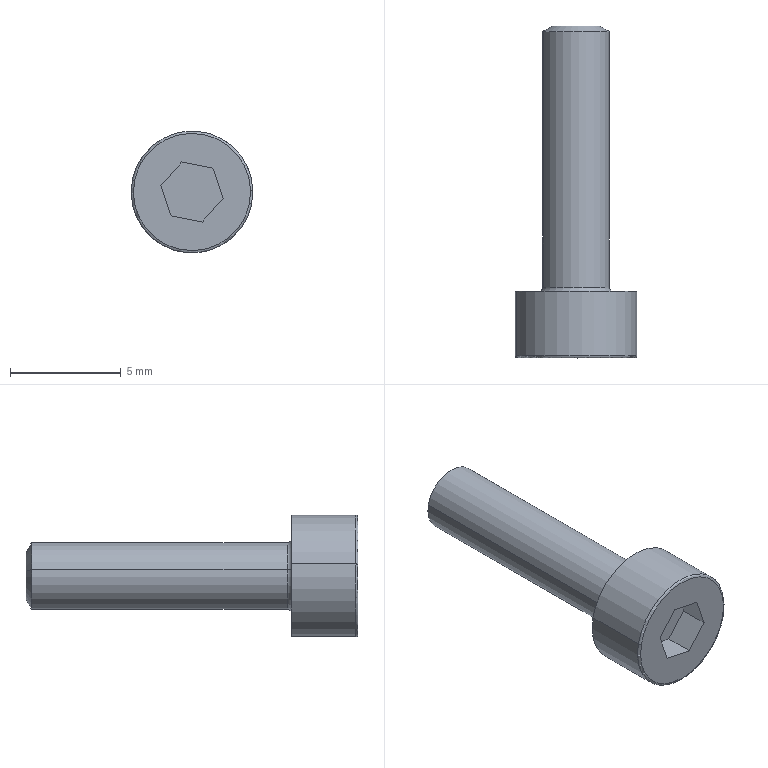Component | SolidWorks | MGL-PACK-01-00WeldedPlate1Assembly-1_SocketHeadCapScrew_M3_12[GB_T70.1-2000]-1 | 1 solid | 20 faces | box 5.5 x 15 x 5.5 mm | volume 149 mm3 | plane 10 | torus 4 | cylinder 4 | cone 2 | commonest cylinder face diameters 5.5 x2 3 x2
STEP:
#1=COLOUR_RGB('',0.7922,0.8196,0.9333);
#2=FILL_AREA_STYLE_COLOUR('',#1);
#3=FILL_AREA_STYLE('',(#2));
#4=SURFACE_STYLE_FILL_AREA(#3);
#5=SURFACE_SIDE_STYLE('',(#4));
#6=SURFACE_STYLE_USAGE(.BOTH.,#5);
#7=PRESENTATION_STYLE_ASSIGNMENT((#6));
#8=CARTESIAN_POINT('',(6.195,-2.224,0.3552));
#9=VERTEX_POINT('',#8);
#10=CARTESIAN_POINT('',(6.4,-2.224,0.314));
#11=VERTEX_POINT('',#10);
#12=CARTESIAN_POINT('',(6.297,-2.224,0.3346));
#13=DIRECTION('',(0.,-1.,-0.));
#14=DIRECTION('',(0.9803,0.,-0.1975));
#15=AXIS2_PLACEMENT_3D('',#12,#13,#14);
#16=CIRCLE('',#15,0.1043);
#17=EDGE_CURVE('',#9,#11,#16,.T.);
#18=ORIENTED_EDGE('',*,*,#17,.F.);
#19=CARTESIAN_POINT('',(6.191,-2.22,0.356));
#20=VERTEX_POINT('',#19);
#21=CARTESIAN_POINT('',(6.195,-2.22,0.3552));
#22=DIRECTION('',(-0.1975,0.,-0.9803));
#23=DIRECTION('',(-0.9803,0.,0.1975));
#24=AXIS2_PLACEMENT_3D('',#21,#22,#23);
#25=CIRCLE('',#24,0.003937);
#26=EDGE_CURVE('',#9,#20,#25,.T.);
#27=ORIENTED_EDGE('',*,*,#26,.T.);
#28=CARTESIAN_POINT('',(6.403,-2.22,0.3133));
#29=VERTEX_POINT('',#28);
#30=CARTESIAN_POINT('',(6.297,-2.22,0.3346));
#31=DIRECTION('',(-0.,1.,0.));
#32=DIRECTION('',(0.9803,0.,-0.1975));
#33=AXIS2_PLACEMENT_3D('',#30,#31,#32);
#34=CIRCLE('',#33,0.1083);
#35=EDGE_CURVE('',#29,#20,#34,.T.);
#36=ORIENTED_EDGE('',*,*,#35,.F.);
#37=CARTESIAN_POINT('',(6.4,-2.22,0.314));
#38=DIRECTION('',(0.1975,-0.,0.9803));
#39=DIRECTION('',(0.9803,0.,-0.1975));
#40=AXIS2_PLACEMENT_3D('',#37,#38,#39);
#41=CIRCLE('',#40,0.003937);
#42=EDGE_CURVE('',#11,#29,#41,.T.);
#43=ORIENTED_EDGE('',*,*,#42,.F.);
#44=EDGE_LOOP('',(#18,#27,#36,#43));
#45=FACE_OUTER_BOUND('',#44,.T.);
#46=CARTESIAN_POINT('',(6.297,-2.22,0.3346));
#47=DIRECTION('',(-0.,1.,0.));
#48=DIRECTION('',(0.9803,0.,-0.1975));
#49=AXIS2_PLACEMENT_3D('',#46,#47,#48);
#50=TOROIDAL_SURFACE('',#49,0.1043,0.003937);
#51=ADVANCED_FACE('',(#45),#50,.T.);
#52=CARTESIAN_POINT('',(6.256,-1.634,0.3429));
#53=VERTEX_POINT('',#52);
#54=CARTESIAN_POINT('',(6.338,-1.634,0.3264));
#55=VERTEX_POINT('',#54);
#56=CARTESIAN_POINT('',(6.297,-1.634,0.3346));
#57=DIRECTION('',(0.,-1.,-0.));
#58=DIRECTION('',(-0.9803,0.,0.1975));
#59=AXIS2_PLACEMENT_3D('',#56,#57,#58);
#60=CIRCLE('',#59,0.04201);
#61=EDGE_CURVE('',#53,#55,#60,.T.);
#62=ORIENTED_EDGE('',*,*,#61,.T.);
#63=CARTESIAN_POINT('',(6.355,-1.644,0.323));
#64=VERTEX_POINT('',#63);
#65=CARTESIAN_POINT('',(6.355,-1.644,0.323));
#66=DIRECTION('',(0.849,-0.5,-0.171));
#67=VECTOR('',#66,39.37);
#68=LINE('',#65,#67);
#69=EDGE_CURVE('',#55,#64,#68,.T.);
#70=ORIENTED_EDGE('',*,*,#69,.T.);
#71=CARTESIAN_POINT('',(6.239,-1.644,0.3463));
#72=VERTEX_POINT('',#71);
#73=CARTESIAN_POINT('',(6.297,-1.644,0.3346));
#74=DIRECTION('',(0.,-1.,-0.));
#75=DIRECTION('',(-0.9803,0.,0.1975));
#76=AXIS2_PLACEMENT_3D('',#73,#74,#75);
#77=CIRCLE('',#76,0.05906);
#78=EDGE_CURVE('',#72,#64,#77,.T.);
#79=ORIENTED_EDGE('',*,*,#78,.F.);
#80=CARTESIAN_POINT('',(6.239,-1.644,0.3463));
#81=DIRECTION('',(-0.849,-0.5,0.171));
#82=VECTOR('',#81,39.37);
#83=LINE('',#80,#82);
#84=EDGE_CURVE('',#53,#72,#83,.T.);
#85=ORIENTED_EDGE('',*,*,#84,.F.);
#86=EDGE_LOOP('',(#62,#70,#79,#85));
#87=FACE_OUTER_BOUND('',#86,.T.);
#88=CARTESIAN_POINT('',(6.297,-1.644,0.3346));
#89=DIRECTION('',(0.,-1.,-0.));
#90=DIRECTION('',(-0.9803,0.,0.1975));
#91=AXIS2_PLACEMENT_3D('',#88,#89,#90);
#92=CONICAL_SURFACE('',#91,0.05906,1.047);
#93=ADVANCED_FACE('',(#87),#92,.T.);
#94=CARTESIAN_POINT('',(6.363,-2.106,0.3214));
#95=VERTEX_POINT('',#94);
#96=CARTESIAN_POINT('',(6.232,-2.106,0.3479));
#97=VERTEX_POINT('',#96);
#98=CARTESIAN_POINT('',(6.297,-2.106,0.3346));
#99=DIRECTION('',(0.,-1.,-0.));
#100=DIRECTION('',(-0.9803,0.,0.1975));
#101=AXIS2_PLACEMENT_3D('',#98,#99,#100);
#102=CIRCLE('',#101,0.06693);
#103=EDGE_CURVE('',#95,#97,#102,.T.);
#104=ORIENTED_EDGE('',*,*,#103,.F.);
#105=CARTESIAN_POINT('',(6.355,-2.098,0.323));
#106=VERTEX_POINT('',#105);
#107=CARTESIAN_POINT('',(6.363,-2.098,0.3214));
#108=DIRECTION('',(-0.1975,0.,-0.9803));
#109=DIRECTION('',(-0.9803,0.,0.1975));
#110=AXIS2_PLACEMENT_3D('',#107,#108,#109);
#111=CIRCLE('',#110,0.007874);
#112=EDGE_CURVE('',#95,#106,#111,.T.);
#113=ORIENTED_EDGE('',*,*,#112,.T.);
#114=CARTESIAN_POINT('',(6.239,-2.098,0.3463));
#115=VERTEX_POINT('',#114);
#116=CARTESIAN_POINT('',(6.297,-2.098,0.3346));
#117=DIRECTION('',(0.,-1.,-0.));
#118=DIRECTION('',(-0.9803,0.,0.1975));
#119=AXIS2_PLACEMENT_3D('',#116,#117,#118);
#120=CIRCLE('',#119,0.05906);
#121=EDGE_CURVE('',#106,#115,#120,.T.);
#122=ORIENTED_EDGE('',*,*,#121,.T.);
#123=CARTESIAN_POINT('',(6.232,-2.098,0.3479));
#124=DIRECTION('',(0.1975,-0.,0.9803));
#125=DIRECTION('',(0.9803,0.,-0.1975));
#126=AXIS2_PLACEMENT_3D('',#123,#124,#125);
#127=CIRCLE('',#126,0.007874);
#128=EDGE_CURVE('',#97,#115,#127,.T.);
#129=ORIENTED_EDGE('',*,*,#128,.F.);
#130=EDGE_LOOP('',(#104,#113,#122,#129));
#131=FACE_OUTER_BOUND('',#130,.T.);
#132=CARTESIAN_POINT('',(6.297,-2.098,0.3346));
#133=DIRECTION('',(0.,-1.,-0.));
#134=DIRECTION('',(-0.9803,-0.,0.1975));
#135=AXIS2_PLACEMENT_3D('',#132,#133,#134);
#136=TOROIDAL_SURFACE('',#135,0.06693,0.007874);
#137=ADVANCED_FACE('',(#131),#136,.F.);
#138=CARTESIAN_POINT('',(6.191,-2.106,0.356));
#139=VERTEX_POINT('',#138);
#140=CARTESIAN_POINT('',(6.403,-2.106,0.3133));
#141=VERTEX_POINT('',#140);
#142=CARTESIAN_POINT('',(6.297,-2.106,0.3346));
#143=DIRECTION('',(0.,-1.,-0.));
#144=DIRECTION('',(-0.9803,0.,0.1975));
#145=AXIS2_PLACEMENT_3D('',#142,#143,#144);
#146=CIRCLE('',#145,0.1083);
#147=EDGE_CURVE('',#139,#141,#146,.T.);
#148=ORIENTED_EDGE('',*,*,#147,.T.);
#149=CARTESIAN_POINT('',(6.403,-2.224,0.3133));
#150=DIRECTION('',(0.,-1.,-0.));
#151=VECTOR('',#150,39.37);
#152=LINE('',#149,#151);
#153=EDGE_CURVE('',#141,#29,#152,.T.);
#154=ORIENTED_EDGE('',*,*,#153,.T.);
#155=ORIENTED_EDGE('',*,*,#35,.T.);
#156=CARTESIAN_POINT('',(6.191,-2.224,0.356));
#157=DIRECTION('',(0.,-1.,-0.));
#158=VECTOR('',#157,39.37);
#159=LINE('',#156,#158);
#160=EDGE_CURVE('',#139,#20,#159,.T.);
#161=ORIENTED_EDGE('',*,*,#160,.F.);
#162=EDGE_LOOP('',(#148,#154,#155,#161));
#163=FACE_OUTER_BOUND('',#162,.T.);
#164=CARTESIAN_POINT('',(6.297,-2.224,0.3346));
#165=DIRECTION('',(0.,-1.,-0.));
#166=DIRECTION('',(-0.9803,0.,0.1975));
#167=AXIS2_PLACEMENT_3D('',#164,#165,#166);
#168=CYLINDRICAL_SURFACE('',#167,0.1083);
#169=ADVANCED_FACE('',(#163),#168,.T.);
#170=ORIENTED_EDGE('',*,*,#78,.T.);
#171=CARTESIAN_POINT('',(6.355,-2.224,0.323));
#172=DIRECTION('',(0.,-1.,-0.));
#173=VECTOR('',#172,39.37);
#174=LINE('',#171,#173);
#175=EDGE_CURVE('',#64,#106,#174,.T.);
#176=ORIENTED_EDGE('',*,*,#175,.T.);
#177=CARTESIAN_POINT('',(6.297,-2.098,0.3346));
#178=DIRECTION('',(0.,-1.,-0.));
#179=DIRECTION('',(-0.9803,0.,0.1975));
#180=AXIS2_PLACEMENT_3D('',#177,#178,#179);
#181=CIRCLE('',#180,0.05906);
#182=EDGE_CURVE('',#115,#106,#181,.T.);
#183=ORIENTED_EDGE('',*,*,#182,.F.);
#184=CARTESIAN_POINT('',(6.239,-2.224,0.3463));
#185=DIRECTION('',(0.,-1.,-0.));
#186=VECTOR('',#185,39.37);
#187=LINE('',#184,#186);
#188=EDGE_CURVE('',#72,#115,#187,.T.);
#189=ORIENTED_EDGE('',*,*,#188,.F.);
#190=EDGE_LOOP('',(#170,#176,#183,#189));
#191=FACE_OUTER_BOUND('',#190,.T.);
#192=CARTESIAN_POINT('',(6.297,-2.224,0.3346));
#193=DIRECTION('',(0.,-1.,-0.));
#194=DIRECTION('',(-0.9803,0.,0.1975));
#195=AXIS2_PLACEMENT_3D('',#192,#193,#194);
#196=CYLINDRICAL_SURFACE('',#195,0.05906);
#197=ADVANCED_FACE('',(#191),#196,.T.);
#198=ORIENTED_EDGE('',*,*,#175,.F.);
#199=CARTESIAN_POINT('',(6.297,-1.644,0.3346));
#200=DIRECTION('',(0.,-1.,-0.));
#201=DIRECTION('',(-0.9803,0.,0.1975));
#202=AXIS2_PLACEMENT_3D('',#199,#200,#201);
#203=CIRCLE('',#202,0.05906);
#204=EDGE_CURVE('',#64,#72,#203,.T.);
#205=ORIENTED_EDGE('',*,*,#204,.T.);
#206=ORIENTED_EDGE('',*,*,#188,.T.);
#207=ORIENTED_EDGE('',*,*,#121,.F.);
#208=EDGE_LOOP('',(#198,#205,#206,#207));
#209=FACE_OUTER_BOUND('',#208,.T.);
#210=CARTESIAN_POINT('',(6.297,-2.224,0.3346));
#211=DIRECTION('',(0.,-1.,-0.));
#212=DIRECTION('',(-0.9803,0.,0.1975));
#213=AXIS2_PLACEMENT_3D('',#210,#211,#212);
#214=CYLINDRICAL_SURFACE('',#213,0.05906);
#215=ADVANCED_FACE('',(#209),#214,.T.);
#216=CARTESIAN_POINT('',(6.297,-2.224,0.3346));
#217=DIRECTION('',(0.,-1.,-0.));
#218=DIRECTION('',(0.9803,0.,-0.1975));
#219=AXIS2_PLACEMENT_3D('',#216,#217,#218);
#220=CIRCLE('',#219,0.1043);
#221=EDGE_CURVE('',#11,#9,#220,.T.);
#222=ORIENTED_EDGE('',*,*,#221,.T.);
#223=ORIENTED_EDGE('',*,*,#17,.T.);
#224=EDGE_LOOP('',(#222,#223));
#225=FACE_OUTER_BOUND('',#224,.T.);
#226=CARTESIAN_POINT('',(6.242,-2.224,0.3458));
#227=VERTEX_POINT('',#226);
#228=CARTESIAN_POINT('',(6.26,-2.224,0.2923));
#229=VERTEX_POINT('',#228);
#230=CARTESIAN_POINT('',(6.242,-2.224,0.3458));
#231=DIRECTION('',(0.3192,0.,-0.9477));
#232=VECTOR('',#231,39.37);
#233=LINE('',#230,#232);
#234=EDGE_CURVE('',#227,#229,#233,.T.);
#235=ORIENTED_EDGE('',*,*,#234,.F.);
#236=CARTESIAN_POINT('',(6.279,-2.224,0.3882));
#237=VERTEX_POINT('',#236);
#238=CARTESIAN_POINT('',(6.279,-2.224,0.3882));
#239=DIRECTION('',(-0.6612,0.,-0.7502));
#240=VECTOR('',#239,39.37);
#241=LINE('',#238,#240);
#242=EDGE_CURVE('',#237,#227,#241,.T.);
#243=ORIENTED_EDGE('',*,*,#242,.F.);
#244=CARTESIAN_POINT('',(6.335,-2.224,0.377));
#245=VERTEX_POINT('',#244);
#246=CARTESIAN_POINT('',(6.335,-2.224,0.377));
#247=DIRECTION('',(-0.9803,-0.,0.1975));
#248=VECTOR('',#247,39.37);
#249=LINE('',#246,#248);
#250=EDGE_CURVE('',#245,#237,#249,.T.);
#251=ORIENTED_EDGE('',*,*,#250,.F.);
#252=CARTESIAN_POINT('',(6.353,-2.224,0.3235));
#253=VERTEX_POINT('',#252);
#254=CARTESIAN_POINT('',(6.353,-2.224,0.3235));
#255=DIRECTION('',(-0.3192,-0.,0.9477));
#256=VECTOR('',#255,39.37);
#257=LINE('',#254,#256);
#258=EDGE_CURVE('',#253,#245,#257,.T.);
#259=ORIENTED_EDGE('',*,*,#258,.F.);
#260=CARTESIAN_POINT('',(6.315,-2.224,0.2811));
#261=VERTEX_POINT('',#260);
#262=CARTESIAN_POINT('',(6.315,-2.224,0.2811));
#263=DIRECTION('',(0.6612,-0.,0.7502));
#264=VECTOR('',#263,39.37);
#265=LINE('',#262,#264);
#266=EDGE_CURVE('',#261,#253,#265,.T.);
#267=ORIENTED_EDGE('',*,*,#266,.F.);
#268=CARTESIAN_POINT('',(6.26,-2.224,0.2923));
#269=DIRECTION('',(0.9803,0.,-0.1975));
#270=VECTOR('',#269,39.37);
#271=LINE('',#268,#270);
#272=EDGE_CURVE('',#229,#261,#271,.T.);
#273=ORIENTED_EDGE('',*,*,#272,.F.);
#274=EDGE_LOOP('',(#235,#243,#251,#259,#267,#273));
#275=FACE_BOUND('',#274,.T.);
#276=CARTESIAN_POINT('',(6.297,-2.224,0.3346));
#277=DIRECTION('',(-0.,1.,0.));
#278=DIRECTION('',(0.9803,0.,-0.1975));
#279=AXIS2_PLACEMENT_3D('',#276,#277,#278);
#280=PLANE('',#279);
#281=ADVANCED_FACE('',(#225,#275),#280,.F.);
#282=ORIENTED_EDGE('',*,*,#153,.F.);
#283=CARTESIAN_POINT('',(6.297,-2.106,0.3346));
#284=DIRECTION('',(0.,-1.,-0.));
#285=DIRECTION('',(-0.9803,0.,0.1975));
#286=AXIS2_PLACEMENT_3D('',#283,#284,#285);
#287=CIRCLE('',#286,0.1083);
#288=EDGE_CURVE('',#141,#139,#287,.T.);
#289=ORIENTED_EDGE('',*,*,#288,.T.);
#290=ORIENTED_EDGE('',*,*,#160,.T.);
#291=CARTESIAN_POINT('',(6.297,-2.22,0.3346));
#292=DIRECTION('',(-0.,1.,0.));
#293=DIRECTION('',(0.9803,0.,-0.1975));
#294=AXIS2_PLACEMENT_3D('',#291,#292,#293);
#295=CIRCLE('',#294,0.1083);
#296=EDGE_CURVE('',#20,#29,#295,.T.);
#297=ORIENTED_EDGE('',*,*,#296,.T.);
#298=EDGE_LOOP('',(#282,#289,#290,#297));
#299=FACE_OUTER_BOUND('',#298,.T.);
#300=CARTESIAN_POINT('',(6.297,-2.224,0.3346));
#301=DIRECTION('',(0.,-1.,-0.));
#302=DIRECTION('',(-0.9803,0.,0.1975));
#303=AXIS2_PLACEMENT_3D('',#300,#301,#302);
#304=CYLINDRICAL_SURFACE('',#303,0.1083);
#305=ADVANCED_FACE('',(#299),#304,.T.);
#306=ORIENTED_EDGE('',*,*,#147,.F.);
#307=ORIENTED_EDGE('',*,*,#288,.F.);
#308=EDGE_LOOP('',(#306,#307));
#309=FACE_OUTER_BOUND('',#308,.T.);
#310=CARTESIAN_POINT('',(6.297,-2.106,0.3346));
#311=DIRECTION('',(0.,-1.,-0.));
#312=DIRECTION('',(-0.9803,0.,0.1975));
#313=AXIS2_PLACEMENT_3D('',#310,#311,#312);
#314=CIRCLE('',#313,0.06693);
#315=EDGE_CURVE('',#97,#95,#314,.T.);
#316=ORIENTED_EDGE('',*,*,#315,.T.);
#317=ORIENTED_EDGE('',*,*,#103,.T.);
#318=EDGE_LOOP('',(#316,#317));
#319=FACE_BOUND('',#318,.T.);
#320=CARTESIAN_POINT('',(6.276,-2.106,0.2285));
#321=DIRECTION('',(0.,-1.,-0.));
#322=DIRECTION('',(-0.9803,-0.,0.1975));
#323=AXIS2_PLACEMENT_3D('',#320,#321,#322);
#324=PLANE('',#323);
#325=ADVANCED_FACE('',(#309,#319),#324,.F.);
#326=ORIENTED_EDGE('',*,*,#112,.F.);
#327=ORIENTED_EDGE('',*,*,#315,.F.);
#328=ORIENTED_EDGE('',*,*,#128,.T.);
#329=ORIENTED_EDGE('',*,*,#182,.T.);
#330=EDGE_LOOP('',(#326,#327,#328,#329));
#331=FACE_OUTER_BOUND('',#330,.T.);
#332=CARTESIAN_POINT('',(6.297,-2.098,0.3346));
#333=DIRECTION('',(0.,-1.,-0.));
#334=DIRECTION('',(-0.9803,-0.,0.1975));
#335=AXIS2_PLACEMENT_3D('',#332,#333,#334);
#336=TOROIDAL_SURFACE('',#335,0.06693,0.007874);
#337=ADVANCED_FACE('',(#331),#336,.F.);
#338=ORIENTED_EDGE('',*,*,#242,.T.);
#339=CARTESIAN_POINT('',(6.242,-2.173,0.3458));
#340=VERTEX_POINT('',#339);
#341=CARTESIAN_POINT('',(6.242,-2.173,0.3458));
#342=DIRECTION('',(0.,-1.,-0.));
#343=VECTOR('',#342,39.37);
#344=LINE('',#341,#343);
#345=EDGE_CURVE('',#340,#227,#344,.T.);
#346=ORIENTED_EDGE('',*,*,#345,.F.);
#347=CARTESIAN_POINT('',(6.279,-2.173,0.3882));
#348=VERTEX_POINT('',#347);
#349=CARTESIAN_POINT('',(6.279,-2.173,0.3882));
#350=DIRECTION('',(-0.6612,0.,-0.7502));
#351=VECTOR('',#350,39.37);
#352=LINE('',#349,#351);
#353=EDGE_CURVE('',#348,#340,#352,.T.);
#354=ORIENTED_EDGE('',*,*,#353,.F.);
#355=CARTESIAN_POINT('',(6.279,-2.173,0.3882));
#356=DIRECTION('',(0.,-1.,-0.));
#357=VECTOR('',#356,39.37);
#358=LINE('',#355,#357);
#359=EDGE_CURVE('',#348,#237,#358,.T.);
#360=ORIENTED_EDGE('',*,*,#359,.T.);
#361=EDGE_LOOP('',(#338,#346,#354,#360));
#362=FACE_OUTER_BOUND('',#361,.T.);
#363=CARTESIAN_POINT('',(6.279,-2.173,0.3882));
#364=DIRECTION('',(-0.7502,-0.,0.6612));
#365=DIRECTION('',(0.6612,-0.,0.7502));
#366=AXIS2_PLACEMENT_3D('',#363,#364,#365);
#367=PLANE('',#366);
#368=ADVANCED_FACE('',(#362),#367,.F.);
#369=ORIENTED_EDGE('',*,*,#250,.T.);
#370=ORIENTED_EDGE('',*,*,#359,.F.);
#371=CARTESIAN_POINT('',(6.335,-2.173,0.377));
#372=VERTEX_POINT('',#371);
#373=CARTESIAN_POINT('',(6.335,-2.173,0.377));
#374=DIRECTION('',(-0.9803,-0.,0.1975));
#375=VECTOR('',#374,39.37);
#376=LINE('',#373,#375);
#377=EDGE_CURVE('',#372,#348,#376,.T.);
#378=ORIENTED_EDGE('',*,*,#377,.F.);
#379=CARTESIAN_POINT('',(6.335,-2.173,0.377));
#380=DIRECTION('',(0.,-1.,-0.));
#381=VECTOR('',#380,39.37);
#382=LINE('',#379,#381);
#383=EDGE_CURVE('',#372,#245,#382,.T.);
#384=ORIENTED_EDGE('',*,*,#383,.T.);
#385=EDGE_LOOP('',(#369,#370,#378,#384));
#386=FACE_OUTER_BOUND('',#385,.T.);
#387=CARTESIAN_POINT('',(6.335,-2.173,0.377));
#388=DIRECTION('',(0.1975,-0.,0.9803));
#389=DIRECTION('',(0.9803,0.,-0.1975));
#390=AXIS2_PLACEMENT_3D('',#387,#388,#389);
#391=PLANE('',#390);
#392=ADVANCED_FACE('',(#386),#391,.F.);
#393=ORIENTED_EDGE('',*,*,#258,.T.);
#394=ORIENTED_EDGE('',*,*,#383,.F.);
#395=CARTESIAN_POINT('',(6.353,-2.173,0.3235));
#396=VERTEX_POINT('',#395);
#397=CARTESIAN_POINT('',(6.353,-2.173,0.3235));
#398=DIRECTION('',(-0.3192,-0.,0.9477));
#399=VECTOR('',#398,39.37);
#400=LINE('',#397,#399);
#401=EDGE_CURVE('',#396,#372,#400,.T.);
#402=ORIENTED_EDGE('',*,*,#401,.F.);
#403=CARTESIAN_POINT('',(6.353,-2.173,0.3235));
#404=DIRECTION('',(0.,-1.,-0.));
#405=VECTOR('',#404,39.37);
#406=LINE('',#403,#405);
#407=EDGE_CURVE('',#396,#253,#406,.T.);
#408=ORIENTED_EDGE('',*,*,#407,.T.);
#409=EDGE_LOOP('',(#393,#394,#402,#408));
#410=FACE_OUTER_BOUND('',#409,.T.);
#411=CARTESIAN_POINT('',(6.353,-2.173,0.3235));
#412=DIRECTION('',(0.9477,0.,0.3192));
#413=DIRECTION('',(0.3192,0.,-0.9477));
#414=AXIS2_PLACEMENT_3D('',#411,#412,#413);
#415=PLANE('',#414);
#416=ADVANCED_FACE('',(#410),#415,.F.);
#417=ORIENTED_EDGE('',*,*,#266,.T.);
#418=ORIENTED_EDGE('',*,*,#407,.F.);
#419=CARTESIAN_POINT('',(6.315,-2.173,0.2811));
#420=VERTEX_POINT('',#419);
#421=CARTESIAN_POINT('',(6.315,-2.173,0.2811));
#422=DIRECTION('',(0.6612,-0.,0.7502));
#423=VECTOR('',#422,39.37);
#424=LINE('',#421,#423);
#425=EDGE_CURVE('',#420,#396,#424,.T.);
#426=ORIENTED_EDGE('',*,*,#425,.F.);
#427=CARTESIAN_POINT('',(6.315,-2.173,0.2811));
#428=DIRECTION('',(0.,-1.,-0.));
#429=VECTOR('',#428,39.37);
#430=LINE('',#427,#429);
#431=EDGE_CURVE('',#420,#261,#430,.T.);
#432=ORIENTED_EDGE('',*,*,#431,.T.);
#433=EDGE_LOOP('',(#417,#418,#426,#432));
#434=FACE_OUTER_BOUND('',#433,.T.);
#435=CARTESIAN_POINT('',(6.315,-2.173,0.2811));
#436=DIRECTION('',(0.7502,0.,-0.6612));
#437=DIRECTION('',(-0.6612,0.,-0.7502));
#438=AXIS2_PLACEMENT_3D('',#435,#436,#437);
#439=PLANE('',#438);
#440=ADVANCED_FACE('',(#434),#439,.F.);
#441=ORIENTED_EDGE('',*,*,#272,.T.);
#442=ORIENTED_EDGE('',*,*,#431,.F.);
#443=CARTESIAN_POINT('',(6.26,-2.173,0.2923));
#444=VERTEX_POINT('',#443);
#445=CARTESIAN_POINT('',(6.26,-2.173,0.2923));
#446=DIRECTION('',(0.9803,0.,-0.1975));
#447=VECTOR('',#446,39.37);
#448=LINE('',#445,#447);
#449=EDGE_CURVE('',#444,#420,#448,.T.);
#450=ORIENTED_EDGE('',*,*,#449,.F.);
#451=CARTESIAN_POINT('',(6.26,-2.173,0.2923));
#452=DIRECTION('',(0.,-1.,-0.));
#453=VECTOR('',#452,39.37);
#454=LINE('',#451,#453);
#455=EDGE_CURVE('',#444,#229,#454,.T.);
#456=ORIENTED_EDGE('',*,*,#455,.T.);
#457=EDGE_LOOP('',(#441,#442,#450,#456));
#458=FACE_OUTER_BOUND('',#457,.T.);
#459=CARTESIAN_POINT('',(6.26,-2.173,0.2923));
#460=DIRECTION('',(-0.1975,0.,-0.9803));
#461=DIRECTION('',(-0.9803,-0.,0.1975));
#462=AXIS2_PLACEMENT_3D('',#459,#460,#461);
#463=PLANE('',#462);
#464=ADVANCED_FACE('',(#458),#463,.F.);
#465=ORIENTED_EDGE('',*,*,#234,.T.);
#466=ORIENTED_EDGE('',*,*,#455,.F.);
#467=CARTESIAN_POINT('',(6.242,-2.173,0.3458));
#468=DIRECTION('',(0.3192,0.,-0.9477));
#469=VECTOR('',#468,39.37);
#470=LINE('',#467,#469);
#471=EDGE_CURVE('',#340,#444,#470,.T.);
#472=ORIENTED_EDGE('',*,*,#471,.F.);
#473=ORIENTED_EDGE('',*,*,#345,.T.);
#474=EDGE_LOOP('',(#465,#466,#472,#473));
#475=FACE_OUTER_BOUND('',#474,.T.);
#476=CARTESIAN_POINT('',(6.242,-2.173,0.3458));
#477=DIRECTION('',(-0.9477,-0.,-0.3192));
#478=DIRECTION('',(-0.3192,-0.,0.9477));
#479=AXIS2_PLACEMENT_3D('',#476,#477,#478);
#480=PLANE('',#479);
#481=ADVANCED_FACE('',(#475),#480,.F.);
#482=ORIENTED_EDGE('',*,*,#353,.T.);
#483=ORIENTED_EDGE('',*,*,#471,.T.);
#484=ORIENTED_EDGE('',*,*,#449,.T.);
#485=ORIENTED_EDGE('',*,*,#425,.T.);
#486=ORIENTED_EDGE('',*,*,#401,.T.);
#487=ORIENTED_EDGE('',*,*,#377,.T.);
#488=EDGE_LOOP('',(#482,#483,#484,#485,#486,#487));
#489=FACE_OUTER_BOUND('',#488,.T.);
#490=CARTESIAN_POINT('',(6.279,-2.173,0.3882));
#491=DIRECTION('',(-0.,1.,0.));
#492=DIRECTION('',(0.9803,0.,-0.1975));
#493=AXIS2_PLACEMENT_3D('',#490,#491,#492);
#494=PLANE('',#493);
#495=ADVANCED_FACE('',(#489),#494,.F.);
#496=ORIENTED_EDGE('',*,*,#69,.F.);
#497=CARTESIAN_POINT('',(6.297,-1.634,0.3346));
#498=DIRECTION('',(0.,-1.,-0.));
#499=DIRECTION('',(-0.9803,0.,0.1975));
#500=AXIS2_PLACEMENT_3D('',#497,#498,#499);
#501=CIRCLE('',#500,0.04201);
#502=EDGE_CURVE('',#55,#53,#501,.T.);
#503=ORIENTED_EDGE('',*,*,#502,.T.);
#504=ORIENTED_EDGE('',*,*,#84,.T.);
#505=ORIENTED_EDGE('',*,*,#204,.F.);
#506=EDGE_LOOP('',(#496,#503,#504,#505));
#507=FACE_OUTER_BOUND('',#506,.T.);
#508=CARTESIAN_POINT('',(6.297,-1.644,0.3346));
#509=DIRECTION('',(0.,-1.,-0.));
#510=DIRECTION('',(-0.9803,0.,0.1975));
#511=AXIS2_PLACEMENT_3D('',#508,#509,#510);
#512=CONICAL_SURFACE('',#511,0.05906,1.047);
#513=ADVANCED_FACE('',(#507),#512,.T.);
#514=ORIENTED_EDGE('',*,*,#61,.F.);
#515=ORIENTED_EDGE('',*,*,#502,.F.);
#516=EDGE_LOOP('',(#514,#515));
#517=FACE_OUTER_BOUND('',#516,.T.);
#518=CARTESIAN_POINT('',(6.286,-1.634,0.2768));
#519=DIRECTION('',(0.,-1.,-0.));
#520=DIRECTION('',(-0.9803,-0.,0.1975));
#521=AXIS2_PLACEMENT_3D('',#518,#519,#520);
#522=PLANE('',#521);
#523=ADVANCED_FACE('',(#517),#522,.F.);
#524=ORIENTED_EDGE('',*,*,#26,.F.);
#525=ORIENTED_EDGE('',*,*,#221,.F.);
#526=ORIENTED_EDGE('',*,*,#42,.T.);
#527=ORIENTED_EDGE('',*,*,#296,.F.);
#528=EDGE_LOOP('',(#524,#525,#526,#527));
#529=FACE_OUTER_BOUND('',#528,.T.);
#530=CARTESIAN_POINT('',(6.297,-2.22,0.3346));
#531=DIRECTION('',(-0.,1.,0.));
#532=DIRECTION('',(0.9803,0.,-0.1975));
#533=AXIS2_PLACEMENT_3D('',#530,#531,#532);
#534=TOROIDAL_SURFACE('',#533,0.1043,0.003937);
#535=ADVANCED_FACE('',(#529),#534,.T.);
#536=CLOSED_SHELL('',(#51,#93,#137,#169,#197,#215,#281,#305,#325,#337,#368,#392,#416,#440,#464,#481,#495,#513,#523,#535));
#537=MANIFOLD_SOLID_BREP('',#536);
#538=STYLED_ITEM('',(#7),#537);
#539=(LENGTH_UNIT()NAMED_UNIT(*)SI_UNIT($,.METRE.));
#540=LENGTH_MEASURE_WITH_UNIT(LENGTH_MEASURE(0.0254),#539);
#541=DIMENSIONAL_EXPONENTS(1.,0.,0.,0.,0.,0.,0.);
#542=(CONVERSION_BASED_UNIT('',#540)LENGTH_UNIT()NAMED_UNIT(#541));
#543=UNCERTAINTY_MEASURE_WITH_UNIT(LENGTH_MEASURE(0.00001),#542,'','');
#544=(NAMED_UNIT(*)PLANE_ANGLE_UNIT()SI_UNIT($,.RADIAN.));
#545=(NAMED_UNIT(*)SI_UNIT($,.STERADIAN.)SOLID_ANGLE_UNIT());
#546=(GEOMETRIC_REPRESENTATION_CONTEXT(3)GLOBAL_UNCERTAINTY_ASSIGNED_CONTEXT((#543))GLOBAL_UNIT_ASSIGNED_CONTEXT((#542,#544,#545))REPRESENTATION_CONTEXT('',''));
#547=MECHANICAL_DESIGN_GEOMETRIC_PRESENTATION_REPRESENTATION('',(#538),#546);
#548=CARTESIAN_POINT('',(0.,0.,0.));
#549=DIRECTION('',(0.,0.,1.));
#550=DIRECTION('',(1.,0.,0.));
#551=AXIS2_PLACEMENT_3D('',#548,#549,#550);
#552=(LENGTH_UNIT()NAMED_UNIT(*)SI_UNIT($,.METRE.));
#553=LENGTH_MEASURE_WITH_UNIT(LENGTH_MEASURE(0.0254),#552);
#554=DIMENSIONAL_EXPONENTS(1.,0.,0.,0.,0.,0.,0.);
#555=(CONVERSION_BASED_UNIT('',#553)LENGTH_UNIT()NAMED_UNIT(#554));
#556=UNCERTAINTY_MEASURE_WITH_UNIT(LENGTH_MEASURE(0.00001),#555,'','');
#557=(NAMED_UNIT(*)PLANE_ANGLE_UNIT()SI_UNIT($,.RADIAN.));
#558=(NAMED_UNIT(*)SI_UNIT($,.STERADIAN.)SOLID_ANGLE_UNIT());
#559=(GEOMETRIC_REPRESENTATION_CONTEXT(3)GLOBAL_UNCERTAINTY_ASSIGNED_CONTEXT((#556))GLOBAL_UNIT_ASSIGNED_CONTEXT((#555,#557,#558))REPRESENTATION_CONTEXT('',''));
#560=ADVANCED_BREP_SHAPE_REPRESENTATION('',(#537,#551),#559);
#561=PRESENTATION_LAYER_ASSIGNMENT('','',(#538));